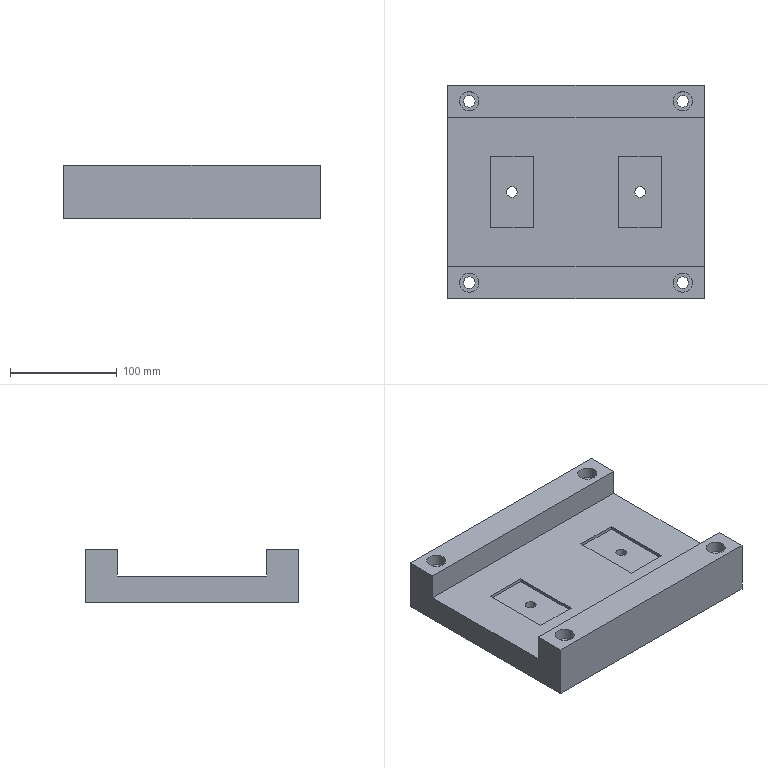Component | NX | SLIDE_TABLE_PART | 1 solid | 34 faces | volume 1514442 mm3 | plane 24 | cylinder 10 | commonest cylinder face diameters 11 x4 18 x4 10 x2